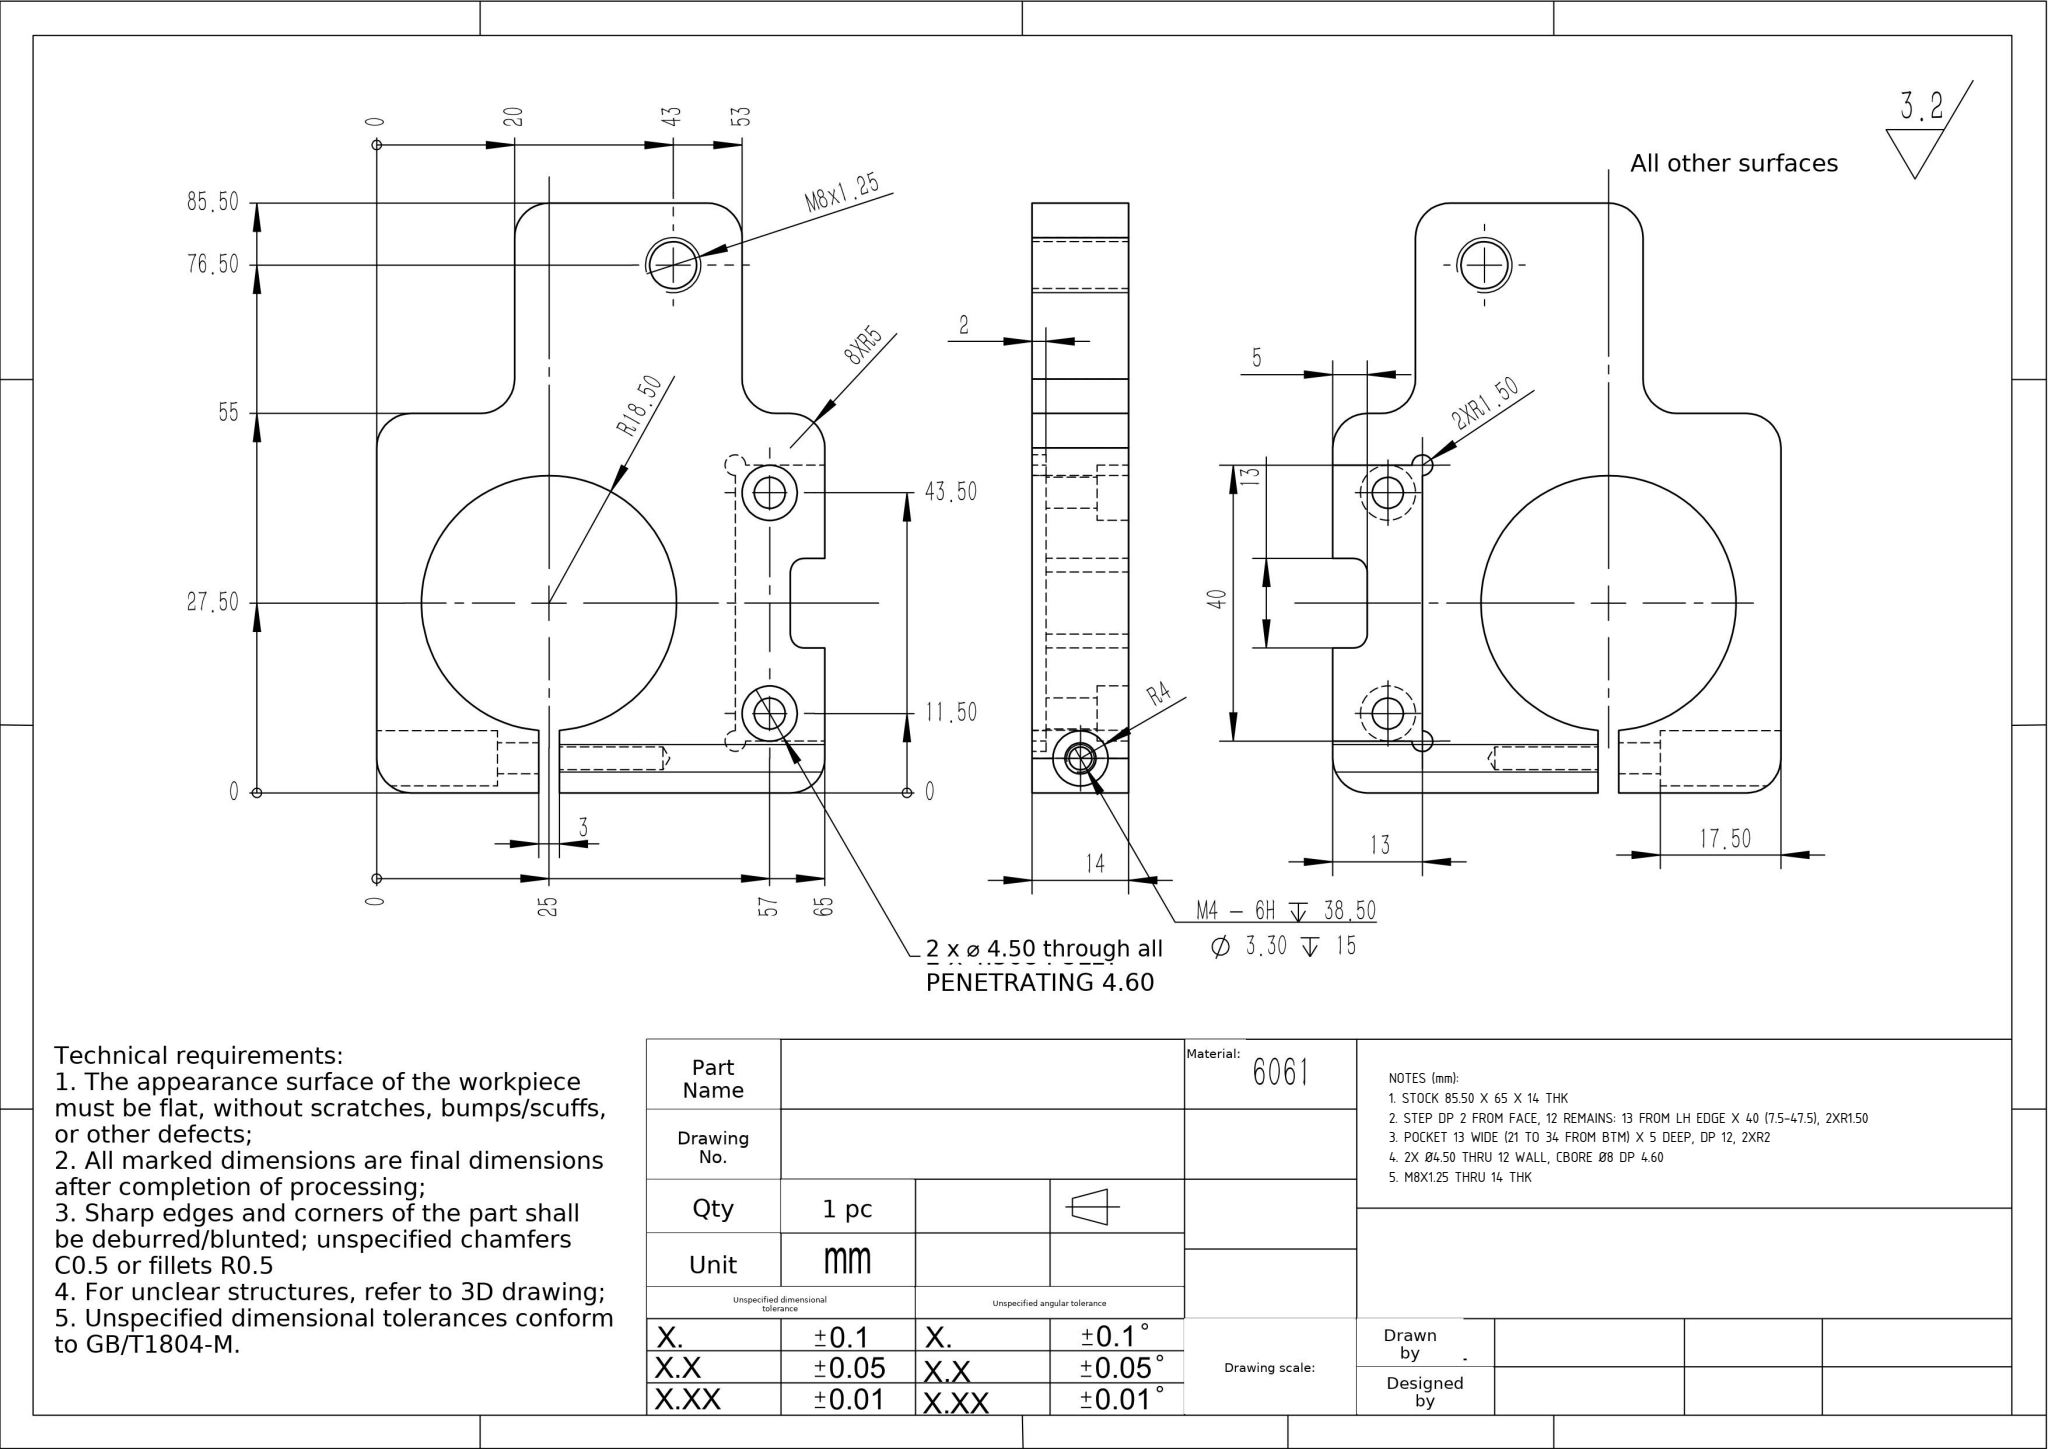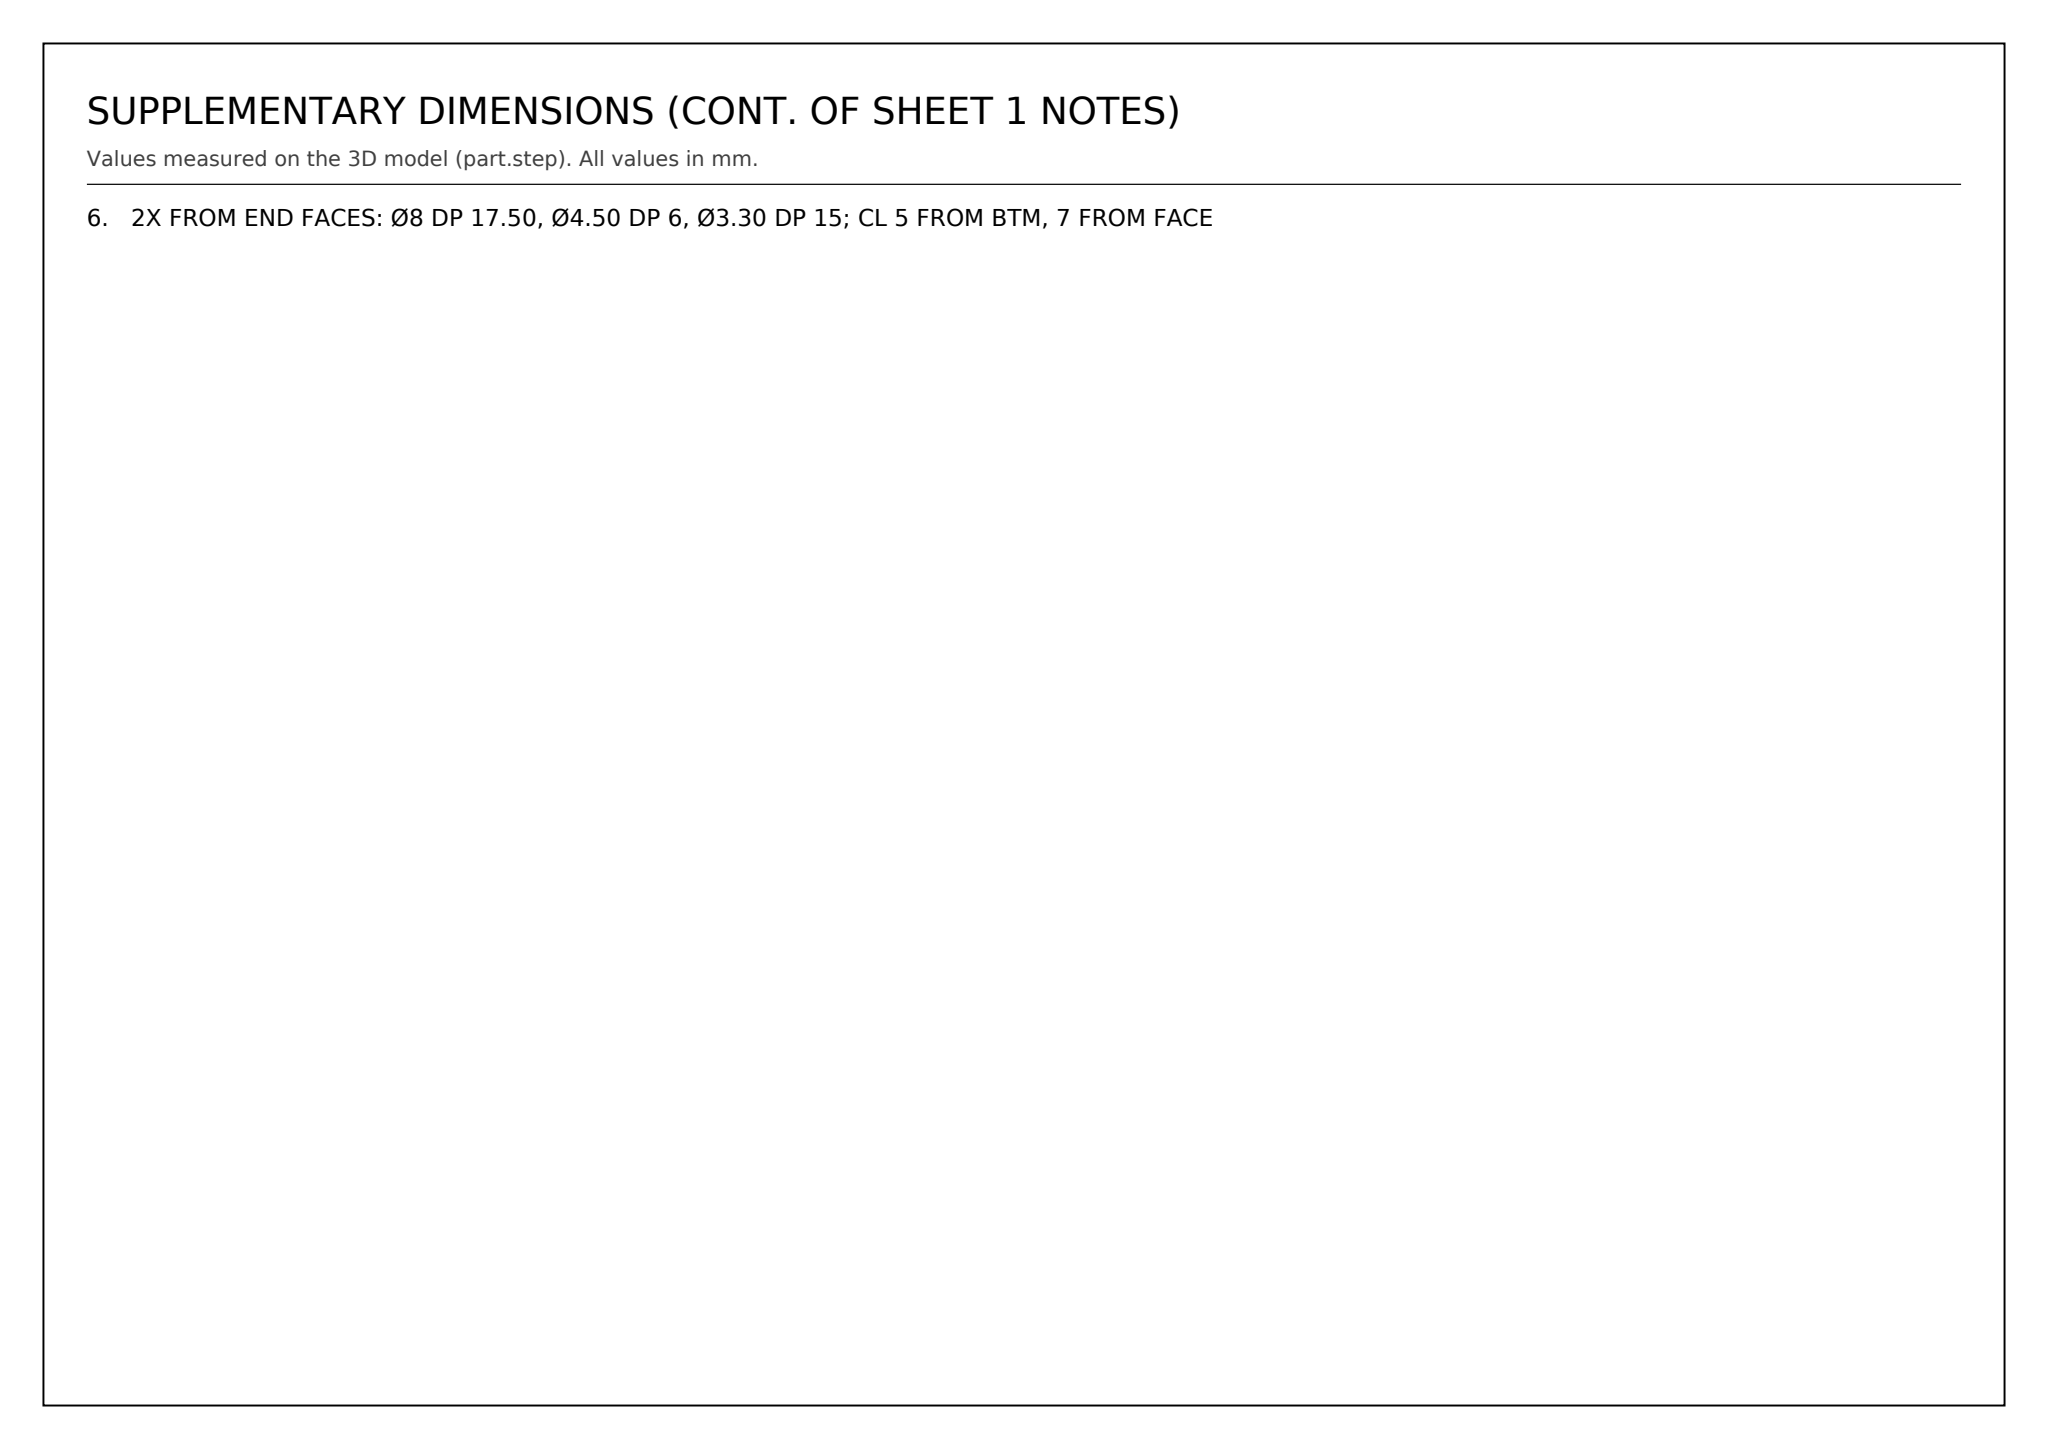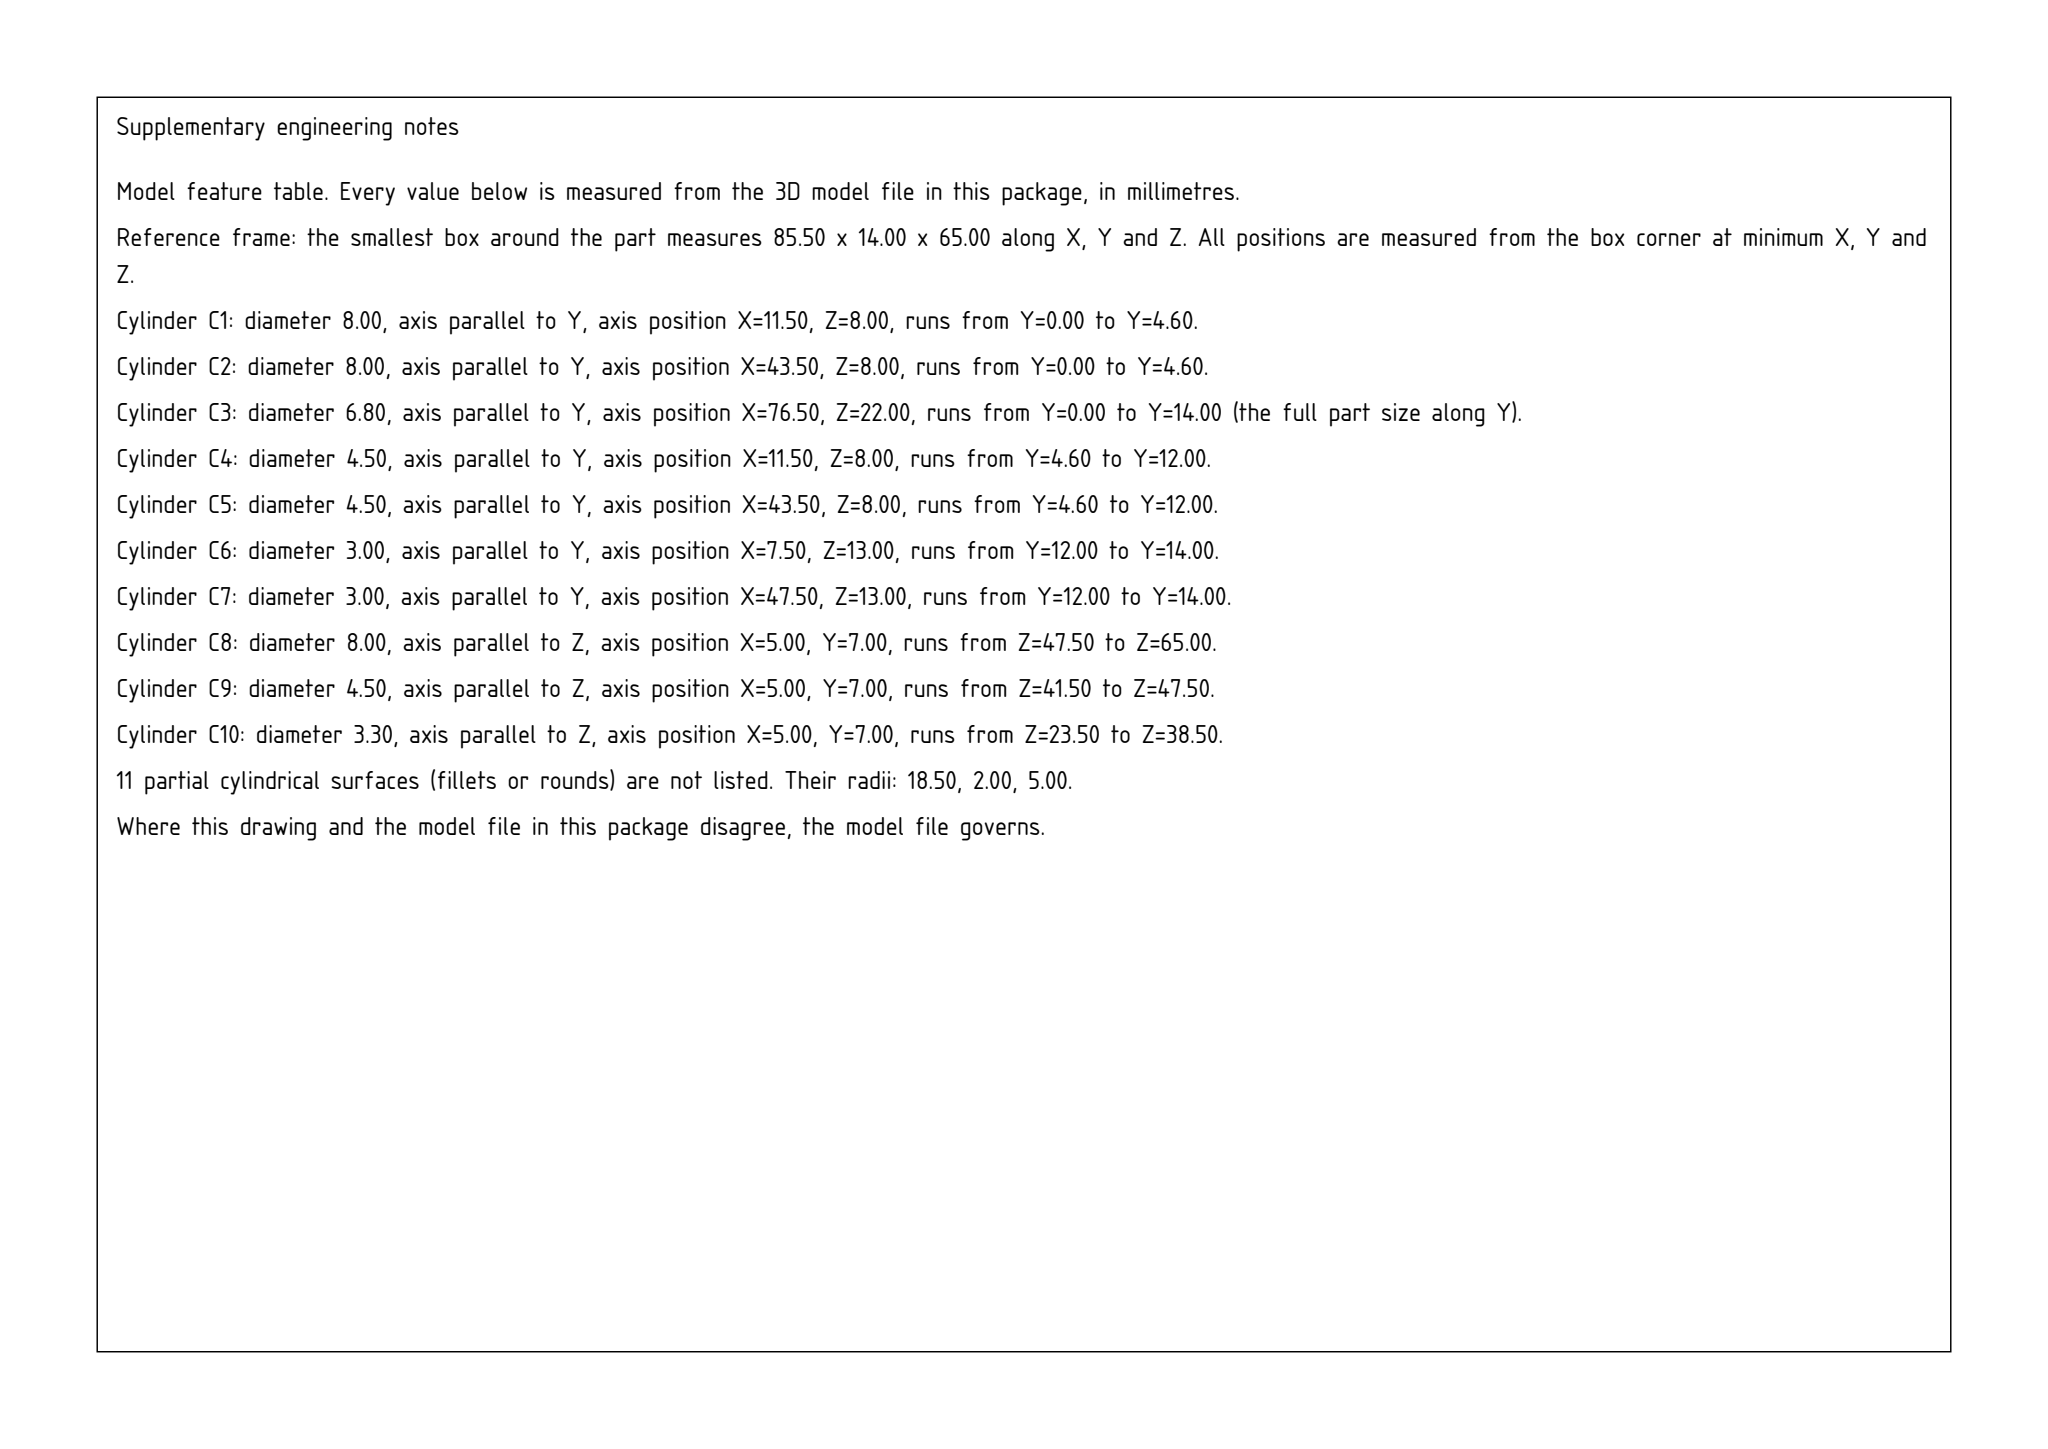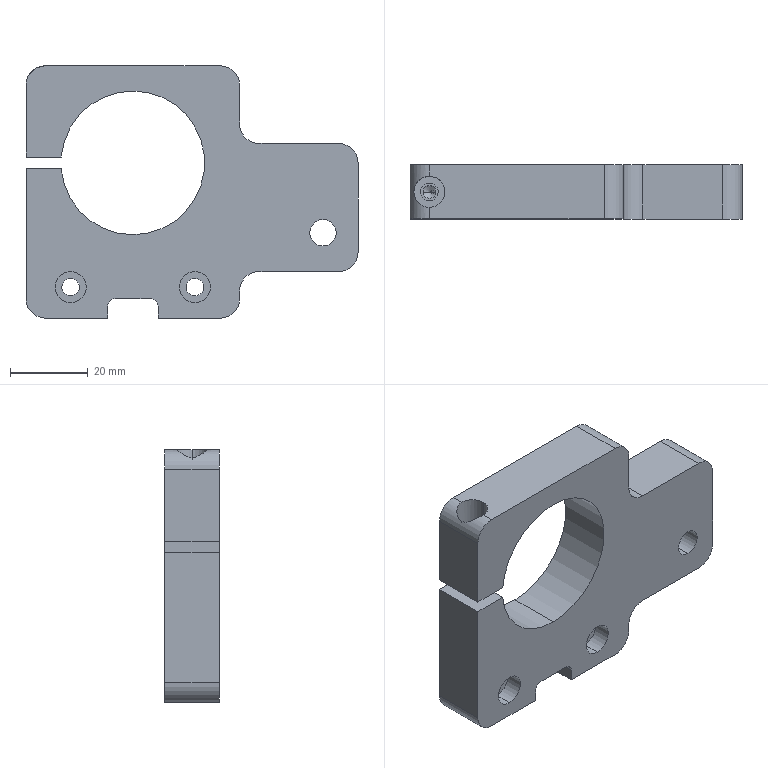Part | SolidWorks | mm | 1 solid | 59 faces | box 85.5 x 14 x 65 mm | volume 44287 mm3 | cylinder 33 | plane 24 | cone 2 | commonest cylinder face diameters 10 x8 4.5 x6 8 x6 3 x4 37 x3 3.3 x2 6.8 x2 4 x2
Drawing notes:
STOCK 85.50 X 65 X 14 THK | from the solid: bbox_xyz 85.5 x 14.0 x 65.0
STEP DP 2 FROM FACE, 12 REMAINS: 13 FROM LH EDGE X 40 (7.5-47.5), 2XR1.50 | from the solid: y-planes 0/4.6/12/14; z=13 bound; R1.50 cyls Ø3 at x7.5 & x47.5, z13 (40 apart)
POCKET 13 WIDE (21 TO 34 FROM BTM) X 5 DEEP, DP 12, 2XR2 | from the solid: x-planes 21 & 34, z-plane 5, R2 corner cyls Ø4 at x=23/32, z=3, L=12
2X Ø4.50 THRU 12 WALL, CBORE Ø8 DP 4.60 | from the solid: coaxial cyls at x=11.5/43.5, z=8: Ø8 L=4.60 over Ø4.50 L=7.40
M8X1.25 THRU 14 THK | from the solid: Ø6.8 y-axis cyl at x=76.5, z=22, L=14 = full thickness
2X FROM END FACES: Ø8 DP 17.50, Ø4.50 DP 6, Ø3.30 DP 15; CL 5 FROM BTM, 7 FROM FACE | from the solid: stacked z-axis cyls on axis x=5, y=7: Ø8 L17.5, Ø4.5 L6, Ø3.3 L15, qty 2; cone 118 ref Ø3.3
build123d program:
from build123d import *

# Parameters (mm, degrees)
BOSS_EXTRUDE1_DEPTH                                = 14
SKETCH2_W                                          = 40
SKETCH2_H                                          = 13
CUT_EXTRUDE1_DEPTH                                 = 2
SKETCH3_R                                          = 1.5
CUT_EXTRUDE2_DEPTH                                 = 2
HOLE_SIZE_ACCORDING_TO_HEX_SOCKET_HEAD_D           = 4.5
HOLE_SIZE_ACCORDING_TO_HEX_SOCKET_HEAD_CBORE_D     = 8
HOLE_SIZE_ACCORDING_TO_HEX_SOCKET_HEAD_CBORE_DEPTH = 4.6
M8X1_25_TAPPED_HOLE1_D                             = 6.8
CUT_EXTRUDE3_REACH                                 = 78.264
SKETCH8_R                                          = 4
SKETCH10_R                                         = 2.25
CUT_EXTRUDE4_DEPTH                                 = 6
M4_TAPPED_HOLE1_D                                  = 3.3
M4_TAPPED_HOLE1_DEPTH                              = 15
M4_TAPPED_HOLE1_TIP                                = 0.9914


with BuildPart() as part:
    # Sketch1 → Boss-Extrude1 (new body)
    with BuildSketch(Plane(origin=(0, 0, 0), x_dir=(1, 0, 0), z_dir=(0, 1, 0))):
        with BuildLine():
            Line((6.5, 40), (6.5, 37))
            ThreePointArc((6.5, 37), (5.914, 35.586), (4.5, 35))
            Line((4.5, 35), (-4.5, 35))
            ThreePointArc((-4.5, 35), (-5.914, 35.586), (-6.5, 37))
            Line((-6.5, 37), (-6.5, 40))
            Line((-6.5, 40), (-22.5, 40))
            ThreePointArc((-22.5, 40), (-26.036, 38.536), (-27.5, 35))
            Line((-27.5, 35), (-27.5, 1.5))
            Line((-27.5, 1.5), (-18.439, 1.5))
            ThreePointArc((-18.439, 1.5), (18.5, 0), (-18.439, -1.5))
            Line((-18.439, -1.5), (-27.5, -1.5))
            Line((-27.5, -1.5), (-27.5, -20))
            ThreePointArc((-27.5, -20), (-26.036, -23.536), (-22.5, -25))
            Line((-22.5, -25), (22.5, -25))
            ThreePointArc((22.5, -25), (26.036, -23.536), (27.5, -20))
            Line((27.5, -20), (27.5, -10))
            ThreePointArc((27.5, -10), (28.964, -6.464), (32.5, -5))
            Line((32.5, -5), (53, -5))
            ThreePointArc((53, -5), (56.536, -3.536), (58, 0))
            Line((58, 0), (58, 23))
            ThreePointArc((58, 23), (56.536, 26.536), (53, 28))
            Line((53, 28), (32.5, 28))
            ThreePointArc((32.5, 28), (28.964, 29.464), (27.5, 33))
            Line((27.5, 33), (27.5, 35))
            ThreePointArc((27.5, 35), (26.036, 38.536), (22.5, 40))
            Line((22.5, 40), (6.5, 40))
        make_face()
    extrude(amount=BOSS_EXTRUDE1_DEPTH)

    # Sketch2 → Cut-Extrude1 (cut)
    with BuildSketch(Plane(origin=(0, 14, 0), x_dir=(1, 0, 0), z_dir=(0, 1, 0))):
        with Locations((0, 33.5)):
            Rectangle(SKETCH2_W, SKETCH2_H)
    extrude(amount=-CUT_EXTRUDE1_DEPTH, mode=Mode.SUBTRACT)

    # Sketch3 → Cut-Extrude2 (cut)
    with BuildSketch(Plane(origin=(0, 14, 0), x_dir=(1, 0, 0), z_dir=(0, 1, 0))):
        with Locations((-20, 27)):
            Circle(SKETCH3_R)
        with Locations((20, 27)):
            Circle(SKETCH3_R)
    extrude(amount=-CUT_EXTRUDE2_DEPTH, mode=Mode.SUBTRACT)

    # Hole Size _according to_ Hex Socket Head (through all)
    with Locations(Plane(origin=(16, 0, -32), x_dir=(0, 0, -1), z_dir=(0, -1, 0))):
        with Locations((0, 0), (0, -32)):
            CounterBoreHole(HOLE_SIZE_ACCORDING_TO_HEX_SOCKET_HEAD_D / 2, HOLE_SIZE_ACCORDING_TO_HEX_SOCKET_HEAD_CBORE_D / 2, HOLE_SIZE_ACCORDING_TO_HEX_SOCKET_HEAD_CBORE_DEPTH)

    # M8x1.25 Tapped Hole1 (through all)
    with Locations(Plane(origin=(49, 0, -18), x_dir=(0, 0, -1), z_dir=(0, -1, 0))):
        with Locations((0, 0)):
            Hole(M8X1_25_TAPPED_HOLE1_D / 2)

    # Sketch8 → Cut-Extrude3 (cut, up to next)
    with BuildSketch(Plane(origin=(0, 0, 7.5), x_dir=(-1, 0, 0), z_dir=(0, 0, -1)), mode=Mode.PRIVATE) as cut_extrude3_sk1:
        with Locations((22.5, 7)):
            Circle(SKETCH8_R)
    cut_extrude3_tool1 = extrude(cut_extrude3_sk1.sketch, amount=-CUT_EXTRUDE3_REACH, mode=Mode.PRIVATE) & part.part
    add(cut_extrude3_tool1.solids().sort_by_distance((-22.5, 7, 7.5))[0], mode=Mode.SUBTRACT)

    # Sketch10 → Cut-Extrude4 (cut)
    with BuildSketch(Plane.XY.offset(7.5)):
        with Locations((-22.5, 7)):
            Circle(SKETCH10_R)
    extrude(amount=-CUT_EXTRUDE4_DEPTH, mode=Mode.SUBTRACT)

    # M4 Tapped Hole1
    with Locations(Plane.XY.offset(-1.5)):
        with Locations((-22.5, 7)):
            Hole(M4_TAPPED_HOLE1_D / 2, depth=M4_TAPPED_HOLE1_DEPTH)
            with Locations((0, 0, -(M4_TAPPED_HOLE1_DEPTH + M4_TAPPED_HOLE1_TIP / 2))):  # 118° drill point
                Cone(0, M4_TAPPED_HOLE1_D / 2, M4_TAPPED_HOLE1_TIP, mode=Mode.SUBTRACT)


solid = part.part